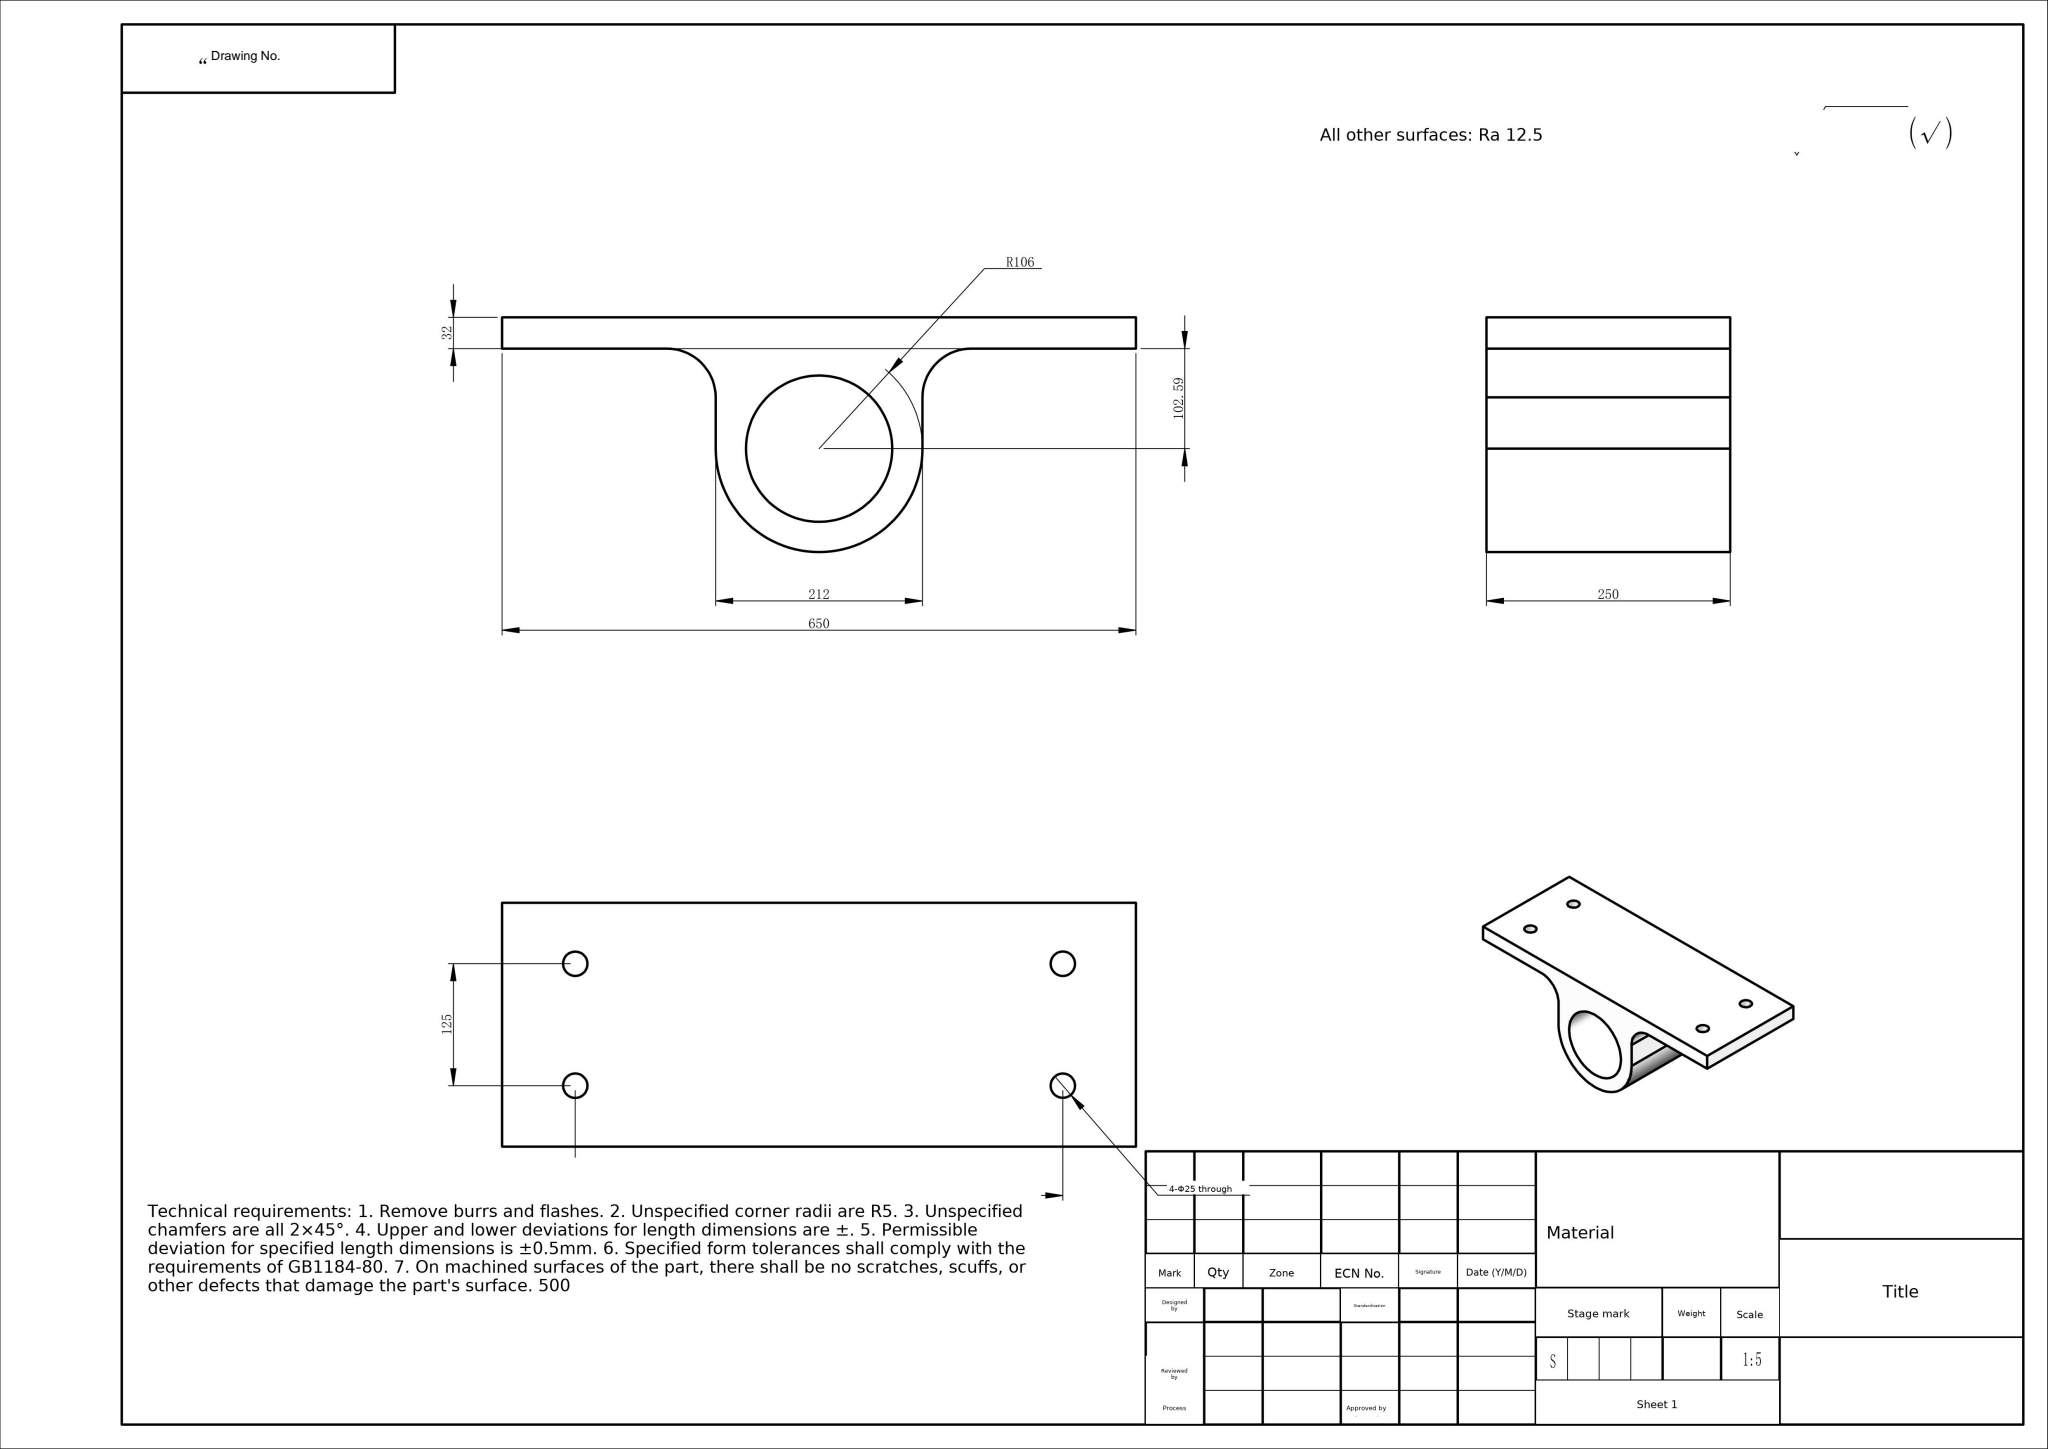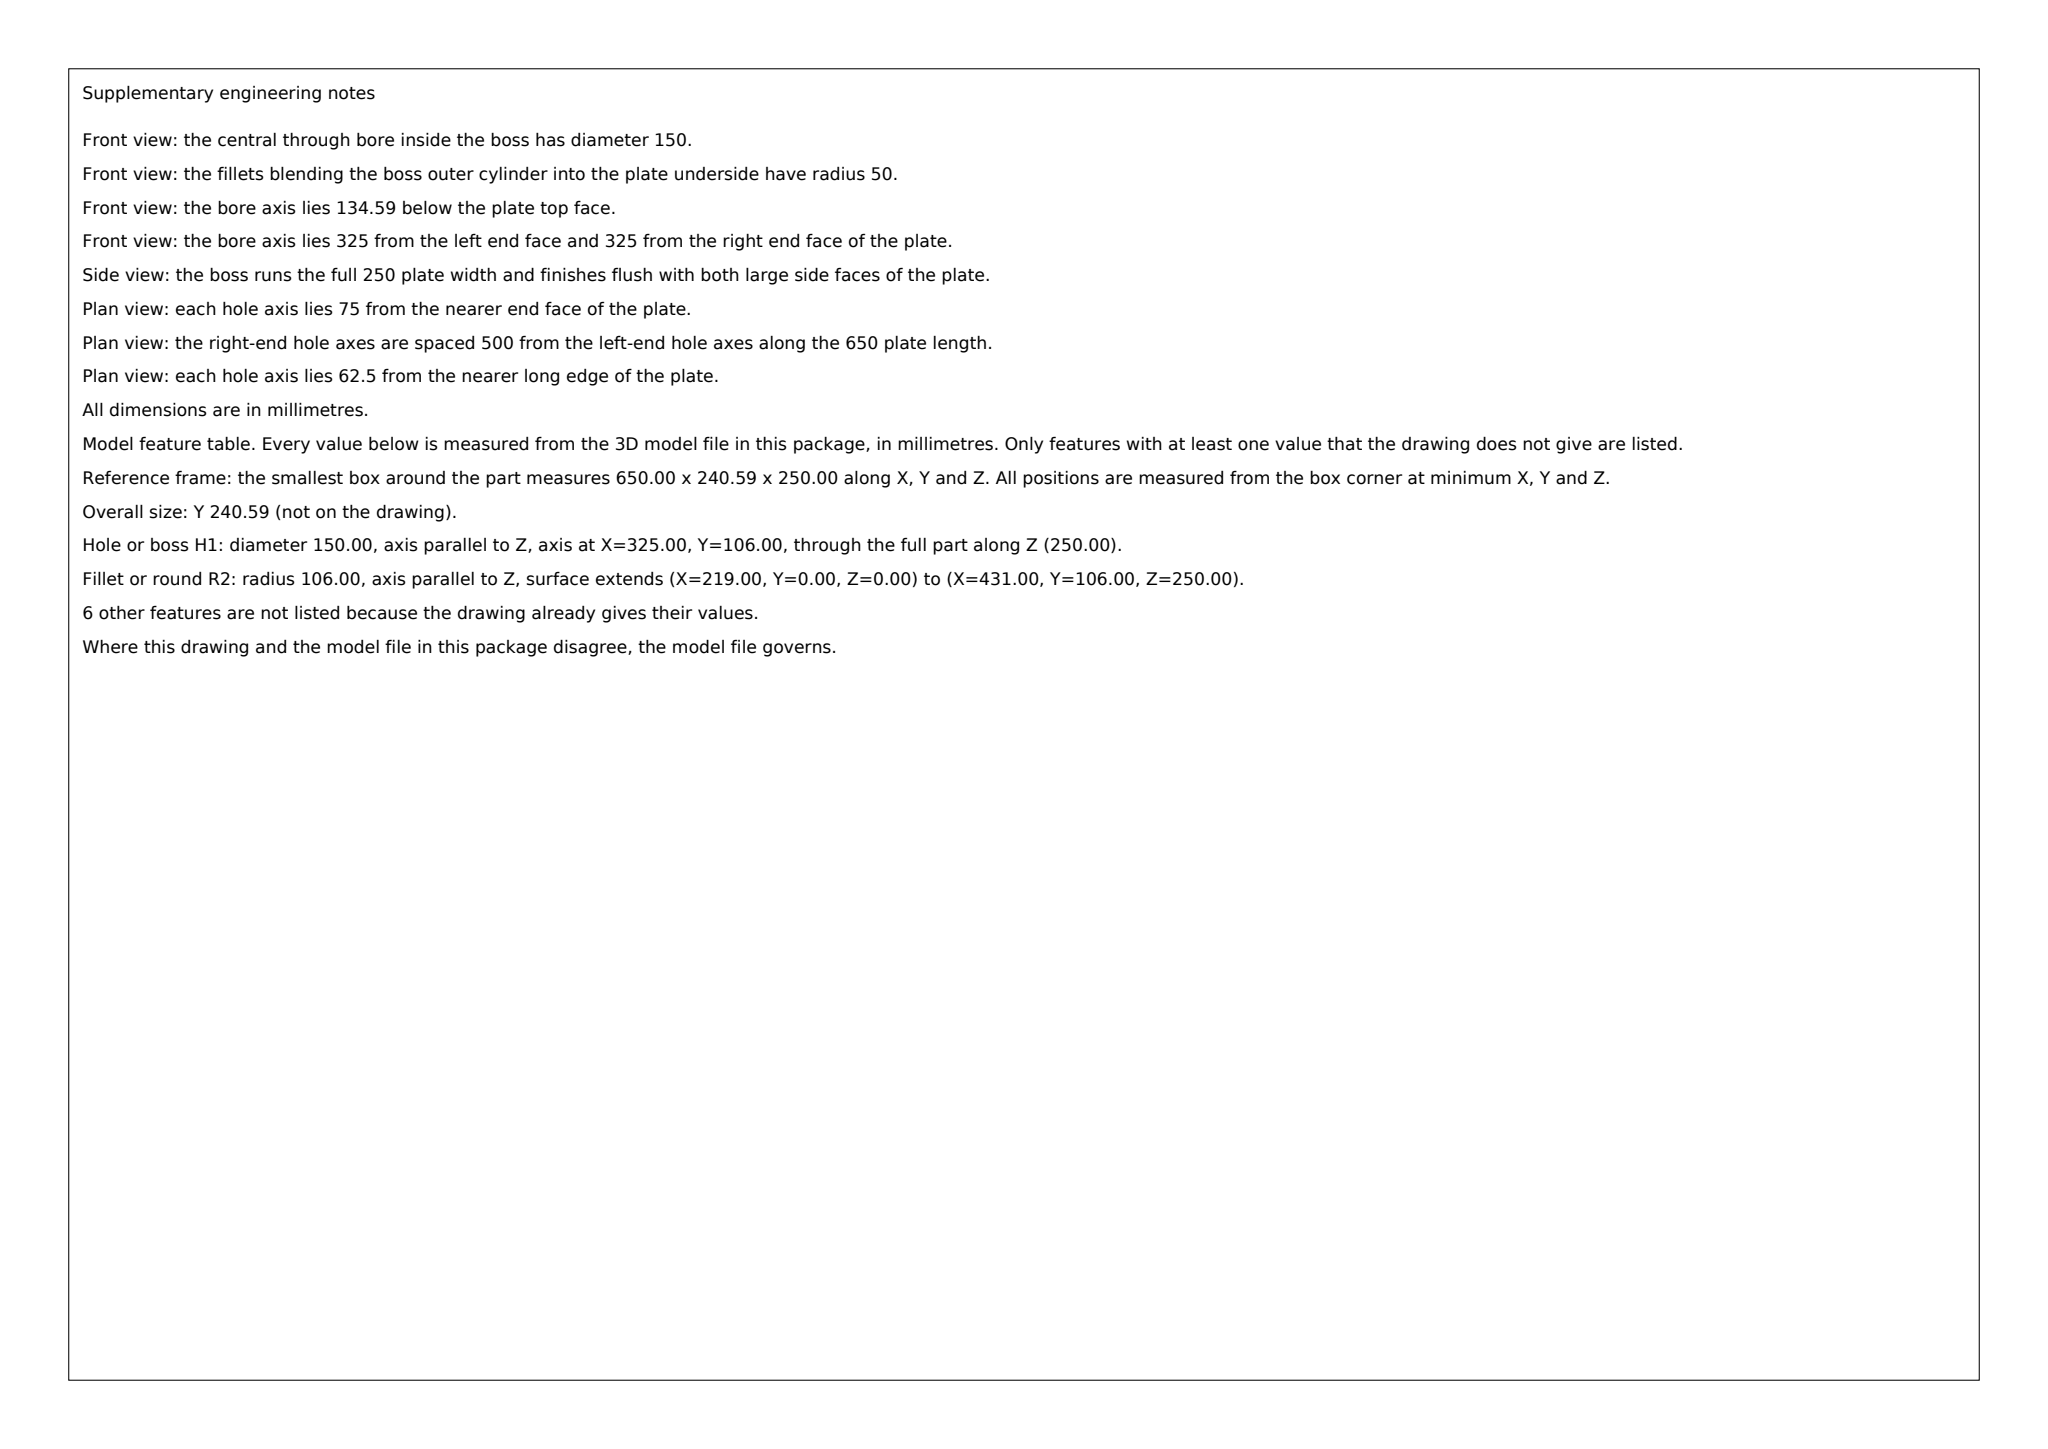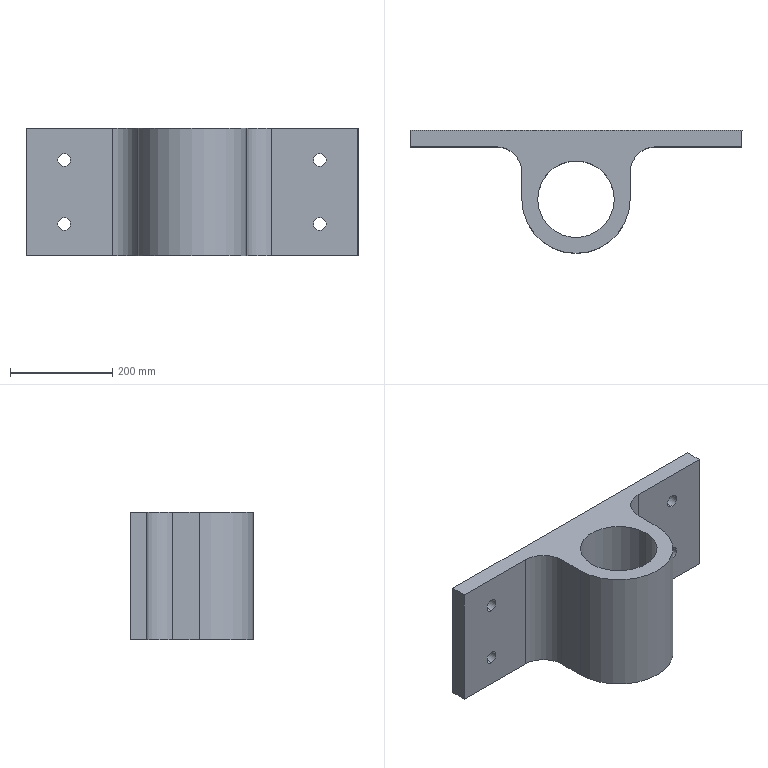Part | SolidWorks | mm | 1 solid | 22 faces | box 650 x 240.59 x 250 mm | volume 10837025 mm3 | cylinder 13 | plane 9 | commonest cylinder face diameters 25 x8 150 x2 100 x2 212 x1
Drawing notes:
Ø150 BORE & R106 BOSS CL 325 FROM LEFT EDGE (CL OF 650) | from the solid: cylinders dia 150 & 212 at x=325.0, bbox x=650.0
UNSPECIFIED LENGTH DIM TOL: ±0.5 | from the solid: Tolerance value not defined in STEP geometry; matched to existing note item 5 (±0.5mm) on drawing; nominal lengths 650 x 240.6 x 250 bbox
build123d program:
from build123d import *

# Parameters (mm, degrees)
SKETCH1_R           = 75
BOSS_EXTRUDE1_DEPTH = 250
SKETCH2_R           = 12.5
CUT_EXTRUDE1_DEPTH  = 250


with BuildPart() as part:
    # Sketch1 → Boss-Extrude1 (new body)
    with BuildSketch(Plane.XY):
        with BuildLine():
            Line((-106, 0), (-106, 52.587))
            ThreePointArc((-106, 52.587), (-120.645, 87.942), (-156, 102.587))
            Line((-156, 102.587), (-325, 102.587))
            Line((-325, 102.587), (-325, 134.587))
            Line((-325, 134.587), (325, 134.587))
            Line((325, 134.587), (325, 102.587))
            Line((325, 102.587), (156, 102.587))
            ThreePointArc((156, 102.587), (120.645, 87.942), (106, 52.587))
            Line((106, 52.587), (106, 0))
            ThreePointArc((106, 0), (0, -106), (-106, 0))
        make_face()
        Circle(SKETCH1_R, mode=Mode.SUBTRACT)
    extrude(amount=BOSS_EXTRUDE1_DEPTH)

    # Sketch2 → Cut-Extrude1 (cut)
    with BuildSketch(Plane(origin=(0, 134.587, 0), x_dir=(1, 0, 0), z_dir=(0, 1, 0))):
        with Locations(Location((-250, -62.5, 0), (0, 0, 270))):
            Circle(SKETCH2_R)
        with Locations(Location((-250, -187.5, 0), (0, 0, 270))):
            Circle(SKETCH2_R)
        with Locations(Location((250, -187.5, 0), (0, 0, 180))):
            Circle(SKETCH2_R)
        with Locations(Location((250, -62.5, 0), (0, 0, 180))):
            Circle(SKETCH2_R)
    extrude(amount=-CUT_EXTRUDE1_DEPTH, mode=Mode.SUBTRACT)


solid = part.part
STEP:
#1=CARTESIAN_POINT('',(250.,102.587,50.));
#2=VERTEX_POINT('',#1);
#3=CARTESIAN_POINT('',(250.,102.587,75.));
#4=VERTEX_POINT('',#3);
#5=CARTESIAN_POINT('',(250.,102.587,62.5));
#6=DIRECTION('',(0.,1.,-0.));
#7=DIRECTION('',(-1.,0.,0.));
#8=AXIS2_PLACEMENT_3D('',#5,#6,#7);
#9=CIRCLE('',#8,12.5);
#10=EDGE_CURVE('',#2,#4,#9,.T.);
#11=ORIENTED_EDGE('',*,*,#10,.F.);
#12=CARTESIAN_POINT('',(250.,134.587,50.));
#13=VERTEX_POINT('',#12);
#14=CARTESIAN_POINT('',(250.,-115.413,50.));
#15=DIRECTION('',(0.,1.,-0.));
#16=VECTOR('',#15,1000.);
#17=LINE('',#14,#16);
#18=EDGE_CURVE('',#2,#13,#17,.T.);
#19=ORIENTED_EDGE('',*,*,#18,.T.);
#20=CARTESIAN_POINT('',(250.,134.587,75.));
#21=VERTEX_POINT('',#20);
#22=CARTESIAN_POINT('',(250.,134.587,62.5));
#23=DIRECTION('',(0.,1.,-0.));
#24=DIRECTION('',(0.,0.,-1.));
#25=AXIS2_PLACEMENT_3D('',#22,#23,#24);
#26=CIRCLE('',#25,12.5);
#27=EDGE_CURVE('',#13,#21,#26,.T.);
#28=ORIENTED_EDGE('',*,*,#27,.T.);
#29=CARTESIAN_POINT('',(250.,-115.413,75.));
#30=DIRECTION('',(0.,1.,-0.));
#31=VECTOR('',#30,1000.);
#32=LINE('',#29,#31);
#33=EDGE_CURVE('',#4,#21,#32,.T.);
#34=ORIENTED_EDGE('',*,*,#33,.F.);
#35=EDGE_LOOP('',(#11,#19,#28,#34));
#36=FACE_OUTER_BOUND('',#35,.T.);
#37=CARTESIAN_POINT('',(250.,-115.413,62.5));
#38=DIRECTION('',(0.,1.,-0.));
#39=DIRECTION('',(0.,0.,1.));
#40=AXIS2_PLACEMENT_3D('',#37,#38,#39);
#41=CYLINDRICAL_SURFACE('',#40,12.5);
#42=ADVANCED_FACE('',(#36),#41,.F.);
#43=CARTESIAN_POINT('',(250.,102.587,175.));
#44=VERTEX_POINT('',#43);
#45=CARTESIAN_POINT('',(250.,102.587,200.));
#46=VERTEX_POINT('',#45);
#47=CARTESIAN_POINT('',(250.,102.587,187.5));
#48=DIRECTION('',(0.,1.,-0.));
#49=DIRECTION('',(-1.,0.,0.));
#50=AXIS2_PLACEMENT_3D('',#47,#48,#49);
#51=CIRCLE('',#50,12.5);
#52=EDGE_CURVE('',#44,#46,#51,.T.);
#53=ORIENTED_EDGE('',*,*,#52,.F.);
#54=CARTESIAN_POINT('',(250.,134.587,175.));
#55=VERTEX_POINT('',#54);
#56=CARTESIAN_POINT('',(250.,-115.413,175.));
#57=DIRECTION('',(0.,1.,-0.));
#58=VECTOR('',#57,1000.);
#59=LINE('',#56,#58);
#60=EDGE_CURVE('',#44,#55,#59,.T.);
#61=ORIENTED_EDGE('',*,*,#60,.T.);
#62=CARTESIAN_POINT('',(250.,134.587,200.));
#63=VERTEX_POINT('',#62);
#64=CARTESIAN_POINT('',(250.,134.587,187.5));
#65=DIRECTION('',(0.,1.,-0.));
#66=DIRECTION('',(0.,0.,-1.));
#67=AXIS2_PLACEMENT_3D('',#64,#65,#66);
#68=CIRCLE('',#67,12.5);
#69=EDGE_CURVE('',#55,#63,#68,.T.);
#70=ORIENTED_EDGE('',*,*,#69,.T.);
#71=CARTESIAN_POINT('',(250.,-115.413,200.));
#72=DIRECTION('',(0.,1.,-0.));
#73=VECTOR('',#72,1000.);
#74=LINE('',#71,#73);
#75=EDGE_CURVE('',#46,#63,#74,.T.);
#76=ORIENTED_EDGE('',*,*,#75,.F.);
#77=EDGE_LOOP('',(#53,#61,#70,#76));
#78=FACE_OUTER_BOUND('',#77,.T.);
#79=CARTESIAN_POINT('',(250.,-115.413,187.5));
#80=DIRECTION('',(0.,1.,-0.));
#81=DIRECTION('',(0.,0.,1.));
#82=AXIS2_PLACEMENT_3D('',#79,#80,#81);
#83=CYLINDRICAL_SURFACE('',#82,12.5);
#84=ADVANCED_FACE('',(#78),#83,.F.);
#85=CARTESIAN_POINT('',(-250.,102.587,175.));
#86=VERTEX_POINT('',#85);
#87=CARTESIAN_POINT('',(-250.,102.587,200.));
#88=VERTEX_POINT('',#87);
#89=CARTESIAN_POINT('',(-250.,102.587,187.5));
#90=DIRECTION('',(-0.,1.,-0.));
#91=DIRECTION('',(-1.,0.,0.));
#92=AXIS2_PLACEMENT_3D('',#89,#90,#91);
#93=CIRCLE('',#92,12.5);
#94=EDGE_CURVE('',#86,#88,#93,.T.);
#95=ORIENTED_EDGE('',*,*,#94,.F.);
#96=CARTESIAN_POINT('',(-250.,134.587,175.));
#97=VERTEX_POINT('',#96);
#98=CARTESIAN_POINT('',(-250.,-115.413,175.));
#99=DIRECTION('',(0.,1.,-0.));
#100=VECTOR('',#99,1000.);
#101=LINE('',#98,#100);
#102=EDGE_CURVE('',#86,#97,#101,.T.);
#103=ORIENTED_EDGE('',*,*,#102,.T.);
#104=CARTESIAN_POINT('',(-250.,134.587,200.));
#105=VERTEX_POINT('',#104);
#106=CARTESIAN_POINT('',(-250.,134.587,187.5));
#107=DIRECTION('',(0.,1.,-0.));
#108=DIRECTION('',(0.,0.,1.));
#109=AXIS2_PLACEMENT_3D('',#106,#107,#108);
#110=CIRCLE('',#109,12.5);
#111=EDGE_CURVE('',#97,#105,#110,.T.);
#112=ORIENTED_EDGE('',*,*,#111,.T.);
#113=CARTESIAN_POINT('',(-250.,-115.413,200.));
#114=DIRECTION('',(0.,1.,-0.));
#115=VECTOR('',#114,1000.);
#116=LINE('',#113,#115);
#117=EDGE_CURVE('',#88,#105,#116,.T.);
#118=ORIENTED_EDGE('',*,*,#117,.F.);
#119=EDGE_LOOP('',(#95,#103,#112,#118));
#120=FACE_OUTER_BOUND('',#119,.T.);
#121=CARTESIAN_POINT('',(-250.,-115.413,187.5));
#122=DIRECTION('',(0.,1.,-0.));
#123=DIRECTION('',(0.,0.,1.));
#124=AXIS2_PLACEMENT_3D('',#121,#122,#123);
#125=CYLINDRICAL_SURFACE('',#124,12.5);
#126=ADVANCED_FACE('',(#120),#125,.F.);
#127=CARTESIAN_POINT('',(-250.,102.587,50.));
#128=VERTEX_POINT('',#127);
#129=CARTESIAN_POINT('',(-250.,102.587,75.));
#130=VERTEX_POINT('',#129);
#131=CARTESIAN_POINT('',(-250.,102.587,62.5));
#132=DIRECTION('',(-0.,1.,-0.));
#133=DIRECTION('',(-1.,0.,0.));
#134=AXIS2_PLACEMENT_3D('',#131,#132,#133);
#135=CIRCLE('',#134,12.5);
#136=EDGE_CURVE('',#128,#130,#135,.T.);
#137=ORIENTED_EDGE('',*,*,#136,.F.);
#138=CARTESIAN_POINT('',(-250.,134.587,50.));
#139=VERTEX_POINT('',#138);
#140=CARTESIAN_POINT('',(-250.,-115.413,50.));
#141=DIRECTION('',(0.,1.,-0.));
#142=VECTOR('',#141,1000.);
#143=LINE('',#140,#142);
#144=EDGE_CURVE('',#128,#139,#143,.T.);
#145=ORIENTED_EDGE('',*,*,#144,.T.);
#146=CARTESIAN_POINT('',(-250.,134.587,75.));
#147=VERTEX_POINT('',#146);
#148=CARTESIAN_POINT('',(-250.,134.587,62.5));
#149=DIRECTION('',(0.,1.,-0.));
#150=DIRECTION('',(0.,0.,1.));
#151=AXIS2_PLACEMENT_3D('',#148,#149,#150);
#152=CIRCLE('',#151,12.5);
#153=EDGE_CURVE('',#139,#147,#152,.T.);
#154=ORIENTED_EDGE('',*,*,#153,.T.);
#155=CARTESIAN_POINT('',(-250.,-115.413,75.));
#156=DIRECTION('',(0.,1.,-0.));
#157=VECTOR('',#156,1000.);
#158=LINE('',#155,#157);
#159=EDGE_CURVE('',#130,#147,#158,.T.);
#160=ORIENTED_EDGE('',*,*,#159,.F.);
#161=EDGE_LOOP('',(#137,#145,#154,#160));
#162=FACE_OUTER_BOUND('',#161,.T.);
#163=CARTESIAN_POINT('',(-250.,-115.413,62.5));
#164=DIRECTION('',(0.,1.,-0.));
#165=DIRECTION('',(0.,0.,1.));
#166=AXIS2_PLACEMENT_3D('',#163,#164,#165);
#167=CYLINDRICAL_SURFACE('',#166,12.5);
#168=ADVANCED_FACE('',(#162),#167,.F.);
#169=CARTESIAN_POINT('',(-75.,0.,250.));
#170=VERTEX_POINT('',#169);
#171=CARTESIAN_POINT('',(75.,0.,250.));
#172=VERTEX_POINT('',#171);
#173=CARTESIAN_POINT('',(0.,0.,250.));
#174=DIRECTION('',(0.,-0.,1.));
#175=DIRECTION('',(1.,0.,0.));
#176=AXIS2_PLACEMENT_3D('',#173,#174,#175);
#177=CIRCLE('',#176,75.);
#178=EDGE_CURVE('',#170,#172,#177,.T.);
#179=ORIENTED_EDGE('',*,*,#178,.T.);
#180=CARTESIAN_POINT('',(75.,0.,0.));
#181=VERTEX_POINT('',#180);
#182=CARTESIAN_POINT('',(75.,0.,250.));
#183=DIRECTION('',(0.,0.,-1.));
#184=VECTOR('',#183,1000.);
#185=LINE('',#182,#184);
#186=EDGE_CURVE('',#172,#181,#185,.T.);
#187=ORIENTED_EDGE('',*,*,#186,.T.);
#188=CARTESIAN_POINT('',(-75.,0.,0.));
#189=VERTEX_POINT('',#188);
#190=CARTESIAN_POINT('',(0.,0.,0.));
#191=DIRECTION('',(0.,-0.,1.));
#192=DIRECTION('',(1.,0.,0.));
#193=AXIS2_PLACEMENT_3D('',#190,#191,#192);
#194=CIRCLE('',#193,75.);
#195=EDGE_CURVE('',#189,#181,#194,.T.);
#196=ORIENTED_EDGE('',*,*,#195,.F.);
#197=CARTESIAN_POINT('',(-75.,0.,250.));
#198=DIRECTION('',(0.,0.,-1.));
#199=VECTOR('',#198,1000.);
#200=LINE('',#197,#199);
#201=EDGE_CURVE('',#170,#189,#200,.T.);
#202=ORIENTED_EDGE('',*,*,#201,.F.);
#203=EDGE_LOOP('',(#179,#187,#196,#202));
#204=FACE_OUTER_BOUND('',#203,.T.);
#205=CARTESIAN_POINT('',(0.,0.,250.));
#206=DIRECTION('',(0.,0.,-1.));
#207=DIRECTION('',(-1.,0.,0.));
#208=AXIS2_PLACEMENT_3D('',#205,#206,#207);
#209=CYLINDRICAL_SURFACE('',#208,75.);
#210=ADVANCED_FACE('',(#204),#209,.F.);
#211=CARTESIAN_POINT('',(-106.,-0.,250.));
#212=VERTEX_POINT('',#211);
#213=CARTESIAN_POINT('',(106.,0.,250.));
#214=VERTEX_POINT('',#213);
#215=CARTESIAN_POINT('',(0.,0.,250.));
#216=DIRECTION('',(0.,-0.,1.));
#217=DIRECTION('',(1.,0.,0.));
#218=AXIS2_PLACEMENT_3D('',#215,#216,#217);
#219=CIRCLE('',#218,106.);
#220=EDGE_CURVE('',#212,#214,#219,.T.);
#221=ORIENTED_EDGE('',*,*,#220,.T.);
#222=CARTESIAN_POINT('',(106.,52.587,250.));
#223=VERTEX_POINT('',#222);
#224=CARTESIAN_POINT('',(106.,0.,250.));
#225=DIRECTION('',(-0.,1.,-0.));
#226=VECTOR('',#225,1000.);
#227=LINE('',#224,#226);
#228=EDGE_CURVE('',#214,#223,#227,.T.);
#229=ORIENTED_EDGE('',*,*,#228,.T.);
#230=CARTESIAN_POINT('',(156.,102.587,250.));
#231=VERTEX_POINT('',#230);
#232=CARTESIAN_POINT('',(156.,52.587,250.));
#233=DIRECTION('',(0.,0.,-1.));
#234=DIRECTION('',(-1.,0.,0.));
#235=AXIS2_PLACEMENT_3D('',#232,#233,#234);
#236=CIRCLE('',#235,50.);
#237=EDGE_CURVE('',#223,#231,#236,.T.);
#238=ORIENTED_EDGE('',*,*,#237,.T.);
#239=CARTESIAN_POINT('',(325.,102.587,250.));
#240=VERTEX_POINT('',#239);
#241=CARTESIAN_POINT('',(156.,102.587,250.));
#242=DIRECTION('',(1.,-0.,-0.));
#243=VECTOR('',#242,1000.);
#244=LINE('',#241,#243);
#245=EDGE_CURVE('',#231,#240,#244,.T.);
#246=ORIENTED_EDGE('',*,*,#245,.T.);
#247=CARTESIAN_POINT('',(325.,134.587,250.));
#248=VERTEX_POINT('',#247);
#249=CARTESIAN_POINT('',(325.,102.587,250.));
#250=DIRECTION('',(0.,1.,-0.));
#251=VECTOR('',#250,1000.);
#252=LINE('',#249,#251);
#253=EDGE_CURVE('',#240,#248,#252,.T.);
#254=ORIENTED_EDGE('',*,*,#253,.T.);
#255=CARTESIAN_POINT('',(-325.,134.587,250.));
#256=VERTEX_POINT('',#255);
#257=CARTESIAN_POINT('',(-325.,134.587,250.));
#258=DIRECTION('',(-1.,0.,0.));
#259=VECTOR('',#258,1000.);
#260=LINE('',#257,#259);
#261=EDGE_CURVE('',#248,#256,#260,.T.);
#262=ORIENTED_EDGE('',*,*,#261,.T.);
#263=CARTESIAN_POINT('',(-325.,102.587,250.));
#264=VERTEX_POINT('',#263);
#265=CARTESIAN_POINT('',(-325.,102.587,250.));
#266=DIRECTION('',(0.,-1.,0.));
#267=VECTOR('',#266,1000.);
#268=LINE('',#265,#267);
#269=EDGE_CURVE('',#256,#264,#268,.T.);
#270=ORIENTED_EDGE('',*,*,#269,.T.);
#271=CARTESIAN_POINT('',(-156.,102.587,250.));
#272=VERTEX_POINT('',#271);
#273=CARTESIAN_POINT('',(-156.,102.587,250.));
#274=DIRECTION('',(1.,0.,-0.));
#275=VECTOR('',#274,1000.);
#276=LINE('',#273,#275);
#277=EDGE_CURVE('',#264,#272,#276,.T.);
#278=ORIENTED_EDGE('',*,*,#277,.T.);
#279=CARTESIAN_POINT('',(-106.,52.587,250.));
#280=VERTEX_POINT('',#279);
#281=CARTESIAN_POINT('',(-156.,52.587,250.));
#282=DIRECTION('',(0.,0.,-1.));
#283=DIRECTION('',(1.,0.,0.));
#284=AXIS2_PLACEMENT_3D('',#281,#282,#283);
#285=CIRCLE('',#284,50.);
#286=EDGE_CURVE('',#272,#280,#285,.T.);
#287=ORIENTED_EDGE('',*,*,#286,.T.);
#288=CARTESIAN_POINT('',(-106.,-0.,250.));
#289=DIRECTION('',(-0.,-1.,0.));
#290=VECTOR('',#289,1000.);
#291=LINE('',#288,#290);
#292=EDGE_CURVE('',#280,#212,#291,.T.);
#293=ORIENTED_EDGE('',*,*,#292,.T.);
#294=EDGE_LOOP('',(#221,#229,#238,#246,#254,#262,#270,#278,#287,#293));
#295=FACE_OUTER_BOUND('',#294,.T.);
#296=ORIENTED_EDGE('',*,*,#178,.F.);
#297=CARTESIAN_POINT('',(0.,0.,250.));
#298=DIRECTION('',(0.,-0.,1.));
#299=DIRECTION('',(1.,0.,0.));
#300=AXIS2_PLACEMENT_3D('',#297,#298,#299);
#301=CIRCLE('',#300,75.);
#302=EDGE_CURVE('',#172,#170,#301,.T.);
#303=ORIENTED_EDGE('',*,*,#302,.F.);
#304=EDGE_LOOP('',(#296,#303));
#305=FACE_BOUND('',#304,.T.);
#306=CARTESIAN_POINT('',(0.,0.,250.));
#307=DIRECTION('',(0.,-0.,1.));
#308=DIRECTION('',(1.,0.,0.));
#309=AXIS2_PLACEMENT_3D('',#306,#307,#308);
#310=PLANE('',#309);
#311=ADVANCED_FACE('',(#295,#305),#310,.T.);
#312=CARTESIAN_POINT('',(-106.,-0.,0.));
#313=VERTEX_POINT('',#312);
#314=CARTESIAN_POINT('',(106.,0.,0.));
#315=VERTEX_POINT('',#314);
#316=CARTESIAN_POINT('',(0.,0.,0.));
#317=DIRECTION('',(0.,-0.,1.));
#318=DIRECTION('',(1.,0.,0.));
#319=AXIS2_PLACEMENT_3D('',#316,#317,#318);
#320=CIRCLE('',#319,106.);
#321=EDGE_CURVE('',#313,#315,#320,.T.);
#322=ORIENTED_EDGE('',*,*,#321,.F.);
#323=CARTESIAN_POINT('',(-106.,52.587,0.));
#324=VERTEX_POINT('',#323);
#325=CARTESIAN_POINT('',(-106.,-0.,0.));
#326=DIRECTION('',(-0.,-1.,0.));
#327=VECTOR('',#326,1000.);
#328=LINE('',#325,#327);
#329=EDGE_CURVE('',#324,#313,#328,.T.);
#330=ORIENTED_EDGE('',*,*,#329,.F.);
#331=CARTESIAN_POINT('',(-156.,102.587,0.));
#332=VERTEX_POINT('',#331);
#333=CARTESIAN_POINT('',(-156.,52.587,0.));
#334=DIRECTION('',(0.,0.,-1.));
#335=DIRECTION('',(1.,0.,0.));
#336=AXIS2_PLACEMENT_3D('',#333,#334,#335);
#337=CIRCLE('',#336,50.);
#338=EDGE_CURVE('',#332,#324,#337,.T.);
#339=ORIENTED_EDGE('',*,*,#338,.F.);
#340=CARTESIAN_POINT('',(-325.,102.587,0.));
#341=VERTEX_POINT('',#340);
#342=CARTESIAN_POINT('',(-156.,102.587,0.));
#343=DIRECTION('',(1.,0.,-0.));
#344=VECTOR('',#343,1000.);
#345=LINE('',#342,#344);
#346=EDGE_CURVE('',#341,#332,#345,.T.);
#347=ORIENTED_EDGE('',*,*,#346,.F.);
#348=CARTESIAN_POINT('',(-325.,134.587,0.));
#349=VERTEX_POINT('',#348);
#350=CARTESIAN_POINT('',(-325.,102.587,0.));
#351=DIRECTION('',(0.,-1.,0.));
#352=VECTOR('',#351,1000.);
#353=LINE('',#350,#352);
#354=EDGE_CURVE('',#349,#341,#353,.T.);
#355=ORIENTED_EDGE('',*,*,#354,.F.);
#356=CARTESIAN_POINT('',(325.,134.587,0.));
#357=VERTEX_POINT('',#356);
#358=CARTESIAN_POINT('',(-325.,134.587,0.));
#359=DIRECTION('',(-1.,0.,0.));
#360=VECTOR('',#359,1000.);
#361=LINE('',#358,#360);
#362=EDGE_CURVE('',#357,#349,#361,.T.);
#363=ORIENTED_EDGE('',*,*,#362,.F.);
#364=CARTESIAN_POINT('',(325.,102.587,0.));
#365=VERTEX_POINT('',#364);
#366=CARTESIAN_POINT('',(325.,102.587,0.));
#367=DIRECTION('',(0.,1.,-0.));
#368=VECTOR('',#367,1000.);
#369=LINE('',#366,#368);
#370=EDGE_CURVE('',#365,#357,#369,.T.);
#371=ORIENTED_EDGE('',*,*,#370,.F.);
#372=CARTESIAN_POINT('',(156.,102.587,0.));
#373=VERTEX_POINT('',#372);
#374=CARTESIAN_POINT('',(156.,102.587,0.));
#375=DIRECTION('',(1.,-0.,-0.));
#376=VECTOR('',#375,1000.);
#377=LINE('',#374,#376);
#378=EDGE_CURVE('',#373,#365,#377,.T.);
#379=ORIENTED_EDGE('',*,*,#378,.F.);
#380=CARTESIAN_POINT('',(106.,52.587,0.));
#381=VERTEX_POINT('',#380);
#382=CARTESIAN_POINT('',(156.,52.587,0.));
#383=DIRECTION('',(0.,0.,-1.));
#384=DIRECTION('',(-1.,0.,0.));
#385=AXIS2_PLACEMENT_3D('',#382,#383,#384);
#386=CIRCLE('',#385,50.);
#387=EDGE_CURVE('',#381,#373,#386,.T.);
#388=ORIENTED_EDGE('',*,*,#387,.F.);
#389=CARTESIAN_POINT('',(106.,0.,0.));
#390=DIRECTION('',(-0.,1.,-0.));
#391=VECTOR('',#390,1000.);
#392=LINE('',#389,#391);
#393=EDGE_CURVE('',#315,#381,#392,.T.);
#394=ORIENTED_EDGE('',*,*,#393,.F.);
#395=EDGE_LOOP('',(#322,#330,#339,#347,#355,#363,#371,#379,#388,#394));
#396=FACE_OUTER_BOUND('',#395,.T.);
#397=ORIENTED_EDGE('',*,*,#195,.T.);
#398=CARTESIAN_POINT('',(0.,0.,0.));
#399=DIRECTION('',(0.,-0.,1.));
#400=DIRECTION('',(1.,0.,0.));
#401=AXIS2_PLACEMENT_3D('',#398,#399,#400);
#402=CIRCLE('',#401,75.);
#403=EDGE_CURVE('',#181,#189,#402,.T.);
#404=ORIENTED_EDGE('',*,*,#403,.T.);
#405=EDGE_LOOP('',(#397,#404));
#406=FACE_BOUND('',#405,.T.);
#407=CARTESIAN_POINT('',(0.,0.,0.));
#408=DIRECTION('',(0.,-0.,1.));
#409=DIRECTION('',(1.,0.,0.));
#410=AXIS2_PLACEMENT_3D('',#407,#408,#409);
#411=PLANE('',#410);
#412=ADVANCED_FACE('',(#396,#406),#411,.F.);
#413=ORIENTED_EDGE('',*,*,#321,.T.);
#414=CARTESIAN_POINT('',(106.,0.,250.));
#415=DIRECTION('',(0.,0.,-1.));
#416=VECTOR('',#415,1000.);
#417=LINE('',#414,#416);
#418=EDGE_CURVE('',#214,#315,#417,.T.);
#419=ORIENTED_EDGE('',*,*,#418,.F.);
#420=ORIENTED_EDGE('',*,*,#220,.F.);
#421=CARTESIAN_POINT('',(-106.,-0.,250.));
#422=DIRECTION('',(0.,0.,-1.));
#423=VECTOR('',#422,1000.);
#424=LINE('',#421,#423);
#425=EDGE_CURVE('',#212,#313,#424,.T.);
#426=ORIENTED_EDGE('',*,*,#425,.T.);
#427=EDGE_LOOP('',(#413,#419,#420,#426));
#428=FACE_OUTER_BOUND('',#427,.T.);
#429=CARTESIAN_POINT('',(0.,0.,250.));
#430=DIRECTION('',(0.,0.,-1.));
#431=DIRECTION('',(-1.,0.,0.));
#432=AXIS2_PLACEMENT_3D('',#429,#430,#431);
#433=CYLINDRICAL_SURFACE('',#432,106.);
#434=ADVANCED_FACE('',(#428),#433,.T.);
#435=ORIENTED_EDGE('',*,*,#393,.T.);
#436=CARTESIAN_POINT('',(106.,52.587,250.));
#437=DIRECTION('',(0.,0.,-1.));
#438=VECTOR('',#437,1000.);
#439=LINE('',#436,#438);
#440=EDGE_CURVE('',#223,#381,#439,.T.);
#441=ORIENTED_EDGE('',*,*,#440,.F.);
#442=ORIENTED_EDGE('',*,*,#228,.F.);
#443=ORIENTED_EDGE('',*,*,#418,.T.);
#444=EDGE_LOOP('',(#435,#441,#442,#443));
#445=FACE_OUTER_BOUND('',#444,.T.);
#446=CARTESIAN_POINT('',(106.,0.,250.));
#447=DIRECTION('',(-1.,-0.,0.));
#448=DIRECTION('',(0.,-1.,0.));
#449=AXIS2_PLACEMENT_3D('',#446,#447,#448);
#450=PLANE('',#449);
#451=ADVANCED_FACE('',(#445),#450,.F.);
#452=ORIENTED_EDGE('',*,*,#387,.T.);
#453=CARTESIAN_POINT('',(156.,102.587,250.));
#454=DIRECTION('',(0.,0.,-1.));
#455=VECTOR('',#454,1000.);
#456=LINE('',#453,#455);
#457=EDGE_CURVE('',#231,#373,#456,.T.);
#458=ORIENTED_EDGE('',*,*,#457,.F.);
#459=ORIENTED_EDGE('',*,*,#237,.F.);
#460=ORIENTED_EDGE('',*,*,#440,.T.);
#461=EDGE_LOOP('',(#452,#458,#459,#460));
#462=FACE_OUTER_BOUND('',#461,.T.);
#463=CARTESIAN_POINT('',(156.,52.587,250.));
#464=DIRECTION('',(0.,0.,-1.));
#465=DIRECTION('',(-1.,0.,0.));
#466=AXIS2_PLACEMENT_3D('',#463,#464,#465);
#467=CYLINDRICAL_SURFACE('',#466,50.);
#468=ADVANCED_FACE('',(#462),#467,.F.);
#469=CARTESIAN_POINT('',(250.,102.587,62.5));
#470=DIRECTION('',(0.,1.,-0.));
#471=DIRECTION('',(-1.,0.,0.));
#472=AXIS2_PLACEMENT_3D('',#469,#470,#471);
#473=CIRCLE('',#472,12.5);
#474=EDGE_CURVE('',#4,#2,#473,.T.);
#475=ORIENTED_EDGE('',*,*,#474,.T.);
#476=ORIENTED_EDGE('',*,*,#10,.T.);
#477=EDGE_LOOP('',(#475,#476));
#478=FACE_BOUND('',#477,.T.);
#479=CARTESIAN_POINT('',(250.,102.587,187.5));
#480=DIRECTION('',(0.,1.,-0.));
#481=DIRECTION('',(-1.,0.,0.));
#482=AXIS2_PLACEMENT_3D('',#479,#480,#481);
#483=CIRCLE('',#482,12.5);
#484=EDGE_CURVE('',#46,#44,#483,.T.);
#485=ORIENTED_EDGE('',*,*,#484,.T.);
#486=ORIENTED_EDGE('',*,*,#52,.T.);
#487=EDGE_LOOP('',(#485,#486));
#488=FACE_BOUND('',#487,.T.);
#489=ORIENTED_EDGE('',*,*,#378,.T.);
#490=CARTESIAN_POINT('',(325.,102.587,250.));
#491=DIRECTION('',(0.,0.,-1.));
#492=VECTOR('',#491,1000.);
#493=LINE('',#490,#492);
#494=EDGE_CURVE('',#240,#365,#493,.T.);
#495=ORIENTED_EDGE('',*,*,#494,.F.);
#496=ORIENTED_EDGE('',*,*,#245,.F.);
#497=ORIENTED_EDGE('',*,*,#457,.T.);
#498=EDGE_LOOP('',(#489,#495,#496,#497));
#499=FACE_OUTER_BOUND('',#498,.T.);
#500=CARTESIAN_POINT('',(156.,102.587,250.));
#501=DIRECTION('',(0.,1.,-0.));
#502=DIRECTION('',(-1.,0.,0.));
#503=AXIS2_PLACEMENT_3D('',#500,#501,#502);
#504=PLANE('',#503);
#505=ADVANCED_FACE('',(#478,#488,#499),#504,.F.);
#506=ORIENTED_EDGE('',*,*,#370,.T.);
#507=CARTESIAN_POINT('',(325.,134.587,250.));
#508=DIRECTION('',(0.,0.,-1.));
#509=VECTOR('',#508,1000.);
#510=LINE('',#507,#509);
#511=EDGE_CURVE('',#248,#357,#510,.T.);
#512=ORIENTED_EDGE('',*,*,#511,.F.);
#513=ORIENTED_EDGE('',*,*,#253,.F.);
#514=ORIENTED_EDGE('',*,*,#494,.T.);
#515=EDGE_LOOP('',(#506,#512,#513,#514));
#516=FACE_OUTER_BOUND('',#515,.T.);
#517=CARTESIAN_POINT('',(325.,102.587,250.));
#518=DIRECTION('',(-1.,0.,0.));
#519=DIRECTION('',(0.,-0.,1.));
#520=AXIS2_PLACEMENT_3D('',#517,#518,#519);
#521=PLANE('',#520);
#522=ADVANCED_FACE('',(#516),#521,.F.);
#523=CARTESIAN_POINT('',(250.,134.587,62.5));
#524=DIRECTION('',(0.,1.,-0.));
#525=DIRECTION('',(0.,0.,-1.));
#526=AXIS2_PLACEMENT_3D('',#523,#524,#525);
#527=CIRCLE('',#526,12.5);
#528=EDGE_CURVE('',#21,#13,#527,.T.);
#529=ORIENTED_EDGE('',*,*,#528,.F.);
#530=ORIENTED_EDGE('',*,*,#27,.F.);
#531=EDGE_LOOP('',(#529,#530));
#532=FACE_BOUND('',#531,.T.);
#533=CARTESIAN_POINT('',(250.,134.587,187.5));
#534=DIRECTION('',(0.,1.,-0.));
#535=DIRECTION('',(0.,0.,-1.));
#536=AXIS2_PLACEMENT_3D('',#533,#534,#535);
#537=CIRCLE('',#536,12.5);
#538=EDGE_CURVE('',#63,#55,#537,.T.);
#539=ORIENTED_EDGE('',*,*,#538,.F.);
#540=ORIENTED_EDGE('',*,*,#69,.F.);
#541=EDGE_LOOP('',(#539,#540));
#542=FACE_BOUND('',#541,.T.);
#543=CARTESIAN_POINT('',(-250.,134.587,187.5));
#544=DIRECTION('',(0.,1.,-0.));
#545=DIRECTION('',(0.,0.,1.));
#546=AXIS2_PLACEMENT_3D('',#543,#544,#545);
#547=CIRCLE('',#546,12.5);
#548=EDGE_CURVE('',#105,#97,#547,.T.);
#549=ORIENTED_EDGE('',*,*,#548,.F.);
#550=ORIENTED_EDGE('',*,*,#111,.F.);
#551=EDGE_LOOP('',(#549,#550));
#552=FACE_BOUND('',#551,.T.);
#553=CARTESIAN_POINT('',(-250.,134.587,62.5));
#554=DIRECTION('',(0.,1.,-0.));
#555=DIRECTION('',(0.,0.,1.));
#556=AXIS2_PLACEMENT_3D('',#553,#554,#555);
#557=CIRCLE('',#556,12.5);
#558=EDGE_CURVE('',#147,#139,#557,.T.);
#559=ORIENTED_EDGE('',*,*,#558,.F.);
#560=ORIENTED_EDGE('',*,*,#153,.F.);
#561=EDGE_LOOP('',(#559,#560));
#562=FACE_BOUND('',#561,.T.);
#563=ORIENTED_EDGE('',*,*,#362,.T.);
#564=CARTESIAN_POINT('',(-325.,134.587,250.));
#565=DIRECTION('',(0.,0.,-1.));
#566=VECTOR('',#565,1000.);
#567=LINE('',#564,#566);
#568=EDGE_CURVE('',#256,#349,#567,.T.);
#569=ORIENTED_EDGE('',*,*,#568,.F.);
#570=ORIENTED_EDGE('',*,*,#261,.F.);
#571=ORIENTED_EDGE('',*,*,#511,.T.);
#572=EDGE_LOOP('',(#563,#569,#570,#571));
#573=FACE_OUTER_BOUND('',#572,.T.);
#574=CARTESIAN_POINT('',(-325.,134.587,250.));
#575=DIRECTION('',(0.,-1.,-0.));
#576=DIRECTION('',(0.,0.,-1.));
#577=AXIS2_PLACEMENT_3D('',#574,#575,#576);
#578=PLANE('',#577);
#579=ADVANCED_FACE('',(#532,#542,#552,#562,#573),#578,.F.);
#580=ORIENTED_EDGE('',*,*,#354,.T.);
#581=CARTESIAN_POINT('',(-325.,102.587,250.));
#582=DIRECTION('',(0.,0.,-1.));
#583=VECTOR('',#582,1000.);
#584=LINE('',#581,#583);
#585=EDGE_CURVE('',#264,#341,#584,.T.);
#586=ORIENTED_EDGE('',*,*,#585,.F.);
#587=ORIENTED_EDGE('',*,*,#269,.F.);
#588=ORIENTED_EDGE('',*,*,#568,.T.);
#589=EDGE_LOOP('',(#580,#586,#587,#588));
#590=FACE_OUTER_BOUND('',#589,.T.);
#591=CARTESIAN_POINT('',(-325.,102.587,250.));
#592=DIRECTION('',(1.,0.,0.));
#593=DIRECTION('',(0.,0.,-1.));
#594=AXIS2_PLACEMENT_3D('',#591,#592,#593);
#595=PLANE('',#594);
#596=ADVANCED_FACE('',(#590),#595,.F.);
#597=CARTESIAN_POINT('',(-250.,102.587,187.5));
#598=DIRECTION('',(-0.,1.,-0.));
#599=DIRECTION('',(-1.,0.,0.));
#600=AXIS2_PLACEMENT_3D('',#597,#598,#599);
#601=CIRCLE('',#600,12.5);
#602=EDGE_CURVE('',#88,#86,#601,.T.);
#603=ORIENTED_EDGE('',*,*,#602,.T.);
#604=ORIENTED_EDGE('',*,*,#94,.T.);
#605=EDGE_LOOP('',(#603,#604));
#606=FACE_BOUND('',#605,.T.);
#607=CARTESIAN_POINT('',(-250.,102.587,62.5));
#608=DIRECTION('',(-0.,1.,-0.));
#609=DIRECTION('',(-1.,0.,0.));
#610=AXIS2_PLACEMENT_3D('',#607,#608,#609);
#611=CIRCLE('',#610,12.5);
#612=EDGE_CURVE('',#130,#128,#611,.T.);
#613=ORIENTED_EDGE('',*,*,#612,.T.);
#614=ORIENTED_EDGE('',*,*,#136,.T.);
#615=EDGE_LOOP('',(#613,#614));
#616=FACE_BOUND('',#615,.T.);
#617=ORIENTED_EDGE('',*,*,#346,.T.);
#618=CARTESIAN_POINT('',(-156.,102.587,250.));
#619=DIRECTION('',(0.,0.,-1.));
#620=VECTOR('',#619,1000.);
#621=LINE('',#618,#620);
#622=EDGE_CURVE('',#272,#332,#621,.T.);
#623=ORIENTED_EDGE('',*,*,#622,.F.);
#624=ORIENTED_EDGE('',*,*,#277,.F.);
#625=ORIENTED_EDGE('',*,*,#585,.T.);
#626=EDGE_LOOP('',(#617,#623,#624,#625));
#627=FACE_OUTER_BOUND('',#626,.T.);
#628=CARTESIAN_POINT('',(-156.,102.587,250.));
#629=DIRECTION('',(-0.,1.,-0.));
#630=DIRECTION('',(-1.,-0.,0.));
#631=AXIS2_PLACEMENT_3D('',#628,#629,#630);
#632=PLANE('',#631);
#633=ADVANCED_FACE('',(#606,#616,#627),#632,.F.);
#634=ORIENTED_EDGE('',*,*,#338,.T.);
#635=CARTESIAN_POINT('',(-106.,52.587,250.));
#636=DIRECTION('',(0.,0.,-1.));
#637=VECTOR('',#636,1000.);
#638=LINE('',#635,#637);
#639=EDGE_CURVE('',#280,#324,#638,.T.);
#640=ORIENTED_EDGE('',*,*,#639,.F.);
#641=ORIENTED_EDGE('',*,*,#286,.F.);
#642=ORIENTED_EDGE('',*,*,#622,.T.);
#643=EDGE_LOOP('',(#634,#640,#641,#642));
#644=FACE_OUTER_BOUND('',#643,.T.);
#645=CARTESIAN_POINT('',(-156.,52.587,250.));
#646=DIRECTION('',(0.,0.,-1.));
#647=DIRECTION('',(-1.,0.,0.));
#648=AXIS2_PLACEMENT_3D('',#645,#646,#647);
#649=CYLINDRICAL_SURFACE('',#648,50.);
#650=ADVANCED_FACE('',(#644),#649,.F.);
#651=ORIENTED_EDGE('',*,*,#329,.T.);
#652=ORIENTED_EDGE('',*,*,#425,.F.);
#653=ORIENTED_EDGE('',*,*,#292,.F.);
#654=ORIENTED_EDGE('',*,*,#639,.T.);
#655=EDGE_LOOP('',(#651,#652,#653,#654));
#656=FACE_OUTER_BOUND('',#655,.T.);
#657=CARTESIAN_POINT('',(-106.,-0.,250.));
#658=DIRECTION('',(1.,-0.,-0.));
#659=DIRECTION('',(0.,1.,-0.));
#660=AXIS2_PLACEMENT_3D('',#657,#658,#659);
#661=PLANE('',#660);
#662=ADVANCED_FACE('',(#656),#661,.F.);
#663=ORIENTED_EDGE('',*,*,#186,.F.);
#664=ORIENTED_EDGE('',*,*,#302,.T.);
#665=ORIENTED_EDGE('',*,*,#201,.T.);
#666=ORIENTED_EDGE('',*,*,#403,.F.);
#667=EDGE_LOOP('',(#663,#664,#665,#666));
#668=FACE_OUTER_BOUND('',#667,.T.);
#669=CARTESIAN_POINT('',(0.,0.,250.));
#670=DIRECTION('',(0.,0.,-1.));
#671=DIRECTION('',(-1.,0.,0.));
#672=AXIS2_PLACEMENT_3D('',#669,#670,#671);
#673=CYLINDRICAL_SURFACE('',#672,75.);
#674=ADVANCED_FACE('',(#668),#673,.F.);
#675=ORIENTED_EDGE('',*,*,#144,.F.);
#676=ORIENTED_EDGE('',*,*,#612,.F.);
#677=ORIENTED_EDGE('',*,*,#159,.T.);
#678=ORIENTED_EDGE('',*,*,#558,.T.);
#679=EDGE_LOOP('',(#675,#676,#677,#678));
#680=FACE_OUTER_BOUND('',#679,.T.);
#681=CARTESIAN_POINT('',(-250.,-115.413,62.5));
#682=DIRECTION('',(0.,1.,-0.));
#683=DIRECTION('',(0.,0.,1.));
#684=AXIS2_PLACEMENT_3D('',#681,#682,#683);
#685=CYLINDRICAL_SURFACE('',#684,12.5);
#686=ADVANCED_FACE('',(#680),#685,.F.);
#687=ORIENTED_EDGE('',*,*,#102,.F.);
#688=ORIENTED_EDGE('',*,*,#602,.F.);
#689=ORIENTED_EDGE('',*,*,#117,.T.);
#690=ORIENTED_EDGE('',*,*,#548,.T.);
#691=EDGE_LOOP('',(#687,#688,#689,#690));
#692=FACE_OUTER_BOUND('',#691,.T.);
#693=CARTESIAN_POINT('',(-250.,-115.413,187.5));
#694=DIRECTION('',(0.,1.,-0.));
#695=DIRECTION('',(0.,0.,1.));
#696=AXIS2_PLACEMENT_3D('',#693,#694,#695);
#697=CYLINDRICAL_SURFACE('',#696,12.5);
#698=ADVANCED_FACE('',(#692),#697,.F.);
#699=ORIENTED_EDGE('',*,*,#60,.F.);
#700=ORIENTED_EDGE('',*,*,#484,.F.);
#701=ORIENTED_EDGE('',*,*,#75,.T.);
#702=ORIENTED_EDGE('',*,*,#538,.T.);
#703=EDGE_LOOP('',(#699,#700,#701,#702));
#704=FACE_OUTER_BOUND('',#703,.T.);
#705=CARTESIAN_POINT('',(250.,-115.413,187.5));
#706=DIRECTION('',(0.,1.,-0.));
#707=DIRECTION('',(0.,0.,1.));
#708=AXIS2_PLACEMENT_3D('',#705,#706,#707);
#709=CYLINDRICAL_SURFACE('',#708,12.5);
#710=ADVANCED_FACE('',(#704),#709,.F.);
#711=ORIENTED_EDGE('',*,*,#18,.F.);
#712=ORIENTED_EDGE('',*,*,#474,.F.);
#713=ORIENTED_EDGE('',*,*,#33,.T.);
#714=ORIENTED_EDGE('',*,*,#528,.T.);
#715=EDGE_LOOP('',(#711,#712,#713,#714));
#716=FACE_OUTER_BOUND('',#715,.T.);
#717=CARTESIAN_POINT('',(250.,-115.413,62.5));
#718=DIRECTION('',(0.,1.,-0.));
#719=DIRECTION('',(0.,0.,1.));
#720=AXIS2_PLACEMENT_3D('',#717,#718,#719);
#721=CYLINDRICAL_SURFACE('',#720,12.5);
#722=ADVANCED_FACE('',(#716),#721,.F.);
#723=CLOSED_SHELL('',(#42,#84,#126,#168,#210,#311,#412,#434,#451,#468,#505,#522,#579,#596,#633,#650,#662,#674,#686,#698,#710,#722));
#724=MANIFOLD_SOLID_BREP('',#723);
#725=CARTESIAN_POINT('',(0.,0.,0.));
#726=DIRECTION('',(0.,0.,1.));
#727=DIRECTION('',(1.,0.,0.));
#728=AXIS2_PLACEMENT_3D('',#725,#726,#727);
#729=(LENGTH_UNIT()NAMED_UNIT(*)SI_UNIT(.MILLI.,.METRE.));
#730=UNCERTAINTY_MEASURE_WITH_UNIT(LENGTH_MEASURE(0.00001),#729,'','');
#731=(NAMED_UNIT(*)PLANE_ANGLE_UNIT()SI_UNIT($,.RADIAN.));
#732=(NAMED_UNIT(*)SI_UNIT($,.STERADIAN.)SOLID_ANGLE_UNIT());
#733=(GEOMETRIC_REPRESENTATION_CONTEXT(3)GLOBAL_UNCERTAINTY_ASSIGNED_CONTEXT((#730))GLOBAL_UNIT_ASSIGNED_CONTEXT((#729,#731,#732))REPRESENTATION_CONTEXT('',''));
#734=ADVANCED_BREP_SHAPE_REPRESENTATION('',(#724,#728),#733);